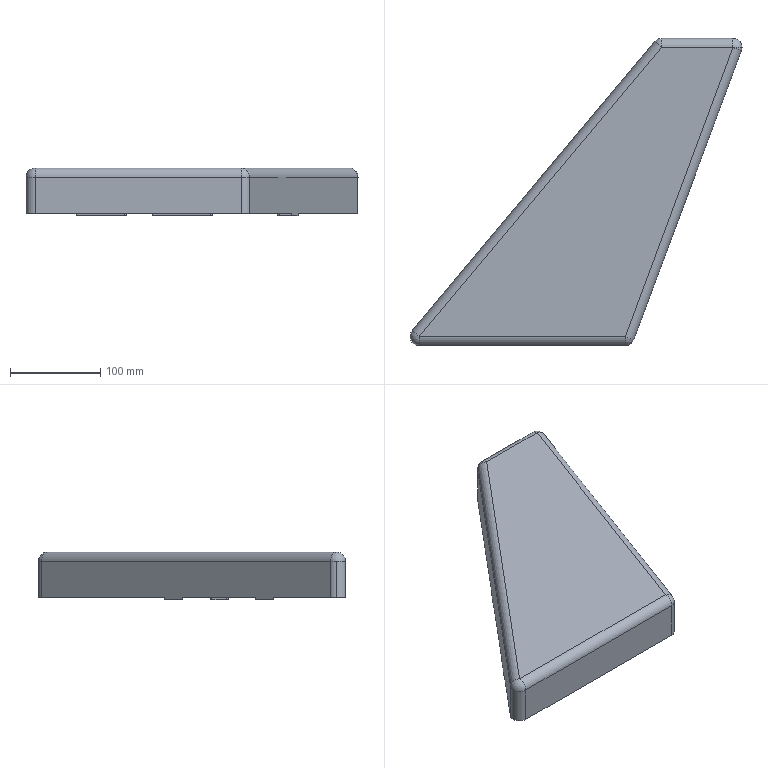Component | SolidWorks | 04-01MotorBracketHousing-1 | 1 solid | 62 faces | volume 226894 mm3 | plane 28 | cylinder 24 | sphere 10 | commonest cylinder face diameters 16 x9 20 x9 4 x6